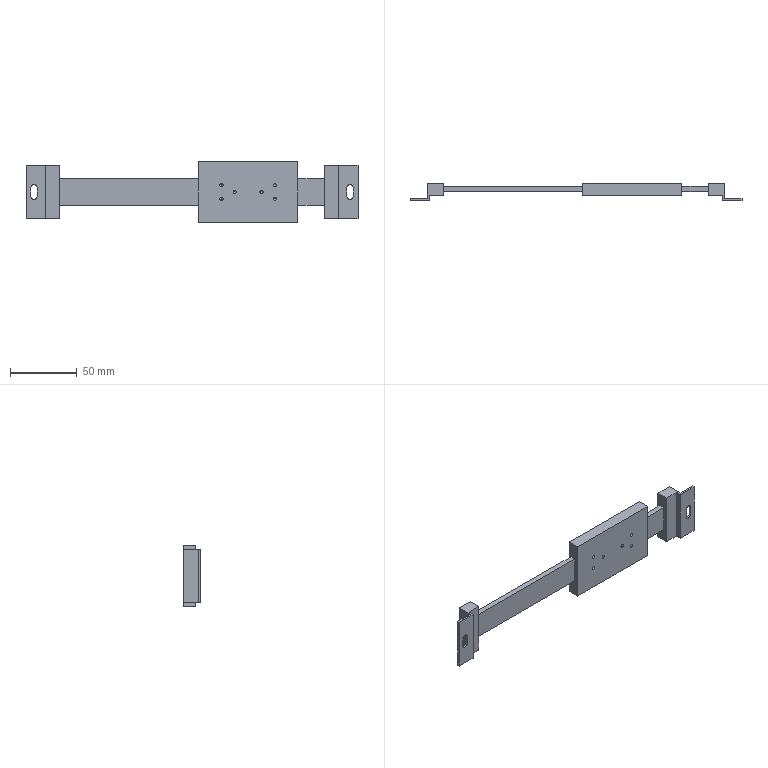Component | SolidWorks | CS021-DigitalScale-Range100-1 | 1 solid | 66 faces | box 248 x 13.25 x 45 mm | volume 50252 mm3 | plane 38 | cylinder 16 | cone 12 | commonest cylinder face diameters 2.5 x12 5 x4 | material AL6061
build123d program:
from build123d import *

# Parameters (mm, degrees)
SKETCH1_W                = 222
SKETCH1_H                = 20
BOSS_EXTRUDE1_DEPTH      = 2
BOSS_EXTRUDE2_DEPTH      = 20
CUT_EXTRUDE1_DEPTH       = 126.961
SKETCH4_W                = 40
SKETCH4_H                = 9
BOSS_EXTRUDE3_DEPTH      = 12
BOSS_EXTRUDE4_DEPTH      = 2
BOSS_EXTRUDE4_DEPTH_BACK = 7
SKETCH5_W                = 74
SKETCH5_H                = 45
M3_TAPPED_HOLE1_D        = 2.5
M3_TAPPED_HOLE1_DEPTH    = 6.5
M3_TAPPED_HOLE1_TIP      = 0.7511


with BuildPart() as part:
    # Sketch1 → Boss-Extrude1 (new, symmetric)
    with BuildSketch(Plane(origin=(0, 0, 0), x_dir=(1, 0, 0), z_dir=(0, 1, 0))):
        Rectangle(SKETCH1_W, SKETCH1_H)
    extrude(amount=BOSS_EXTRUDE1_DEPTH, both=True)

    # Sketch2 → Boss-Extrude2 (add, symmetric)
    with BuildSketch(Plane.XY):
        Polygon((-109.5, -2), (-109.5, -9), (-124, -9), (-124, -7.5), (-111, -7.5), (-111, -2), align=None)
    boss_extrude2 = extrude(amount=BOSS_EXTRUDE2_DEPTH, both=True)

    # Sketch3 → Cut-Extrude1 (cut, through all)
    with BuildSketch(Plane(origin=(0, -7.5, 0), x_dir=(1, 0, 0), z_dir=(0, 1, 0))):
        with BuildLine():
            Line((-115.5, 3), (-115.5, -3))
            ThreePointArc((-115.5, -3), (-118, -5.5), (-120.5, -3))
            Line((-120.5, -3), (-120.5, 3))
            ThreePointArc((-120.5, 3), (-118, 5.5), (-115.5, 3))
        make_face()
    cut_extrude1 = extrude(amount=-CUT_EXTRUDE1_DEPTH, mode=Mode.SUBTRACT)

    # Sketch4 → Boss-Extrude3 (add)
    with BuildSketch(Plane.ZY.offset(111)):
        with Locations((0, -0.25)):
            Rectangle(SKETCH4_W, SKETCH4_H)
    boss_extrude3 = extrude(amount=-BOSS_EXTRUDE3_DEPTH)

    # Mirror1: Boss-Extrude2, Cut-Extrude1, Boss-Extrude3 across plane
    add(boss_extrude2.mirror(Plane(origin=(0, 0, 0), x_dir=(0, 0, 1), z_dir=(1, 0, 0))))
    add(cut_extrude1.mirror(Plane(origin=(0, 0, 0), x_dir=(0, 0, 1), z_dir=(1, 0, 0))), mode=Mode.SUBTRACT)
    add(boss_extrude3.mirror(Plane(origin=(0, 0, 0), x_dir=(0, 0, 1), z_dir=(1, 0, 0))))

    # Sketch5 → Boss-Extrude4 (add, two sides: drawn at the far end of the back side and taken through both)
    with BuildSketch(Plane(origin=(0, 2, 0), x_dir=(1, 0, 0), z_dir=(0, 1, 0)).offset(-BOSS_EXTRUDE4_DEPTH_BACK)):
        with Locations((-42, 0)):
            Rectangle(SKETCH5_W, SKETCH5_H)
    extrude(amount=BOSS_EXTRUDE4_DEPTH + BOSS_EXTRUDE4_DEPTH_BACK)

    # M3 Tapped Hole1
    with Locations(Plane(origin=(0, -5, 0), x_dir=(-1, 0, 0), z_dir=(0, -1, 0))):
        with Locations((52, 0), (32, 0), (22, 5), (22, -5), (62, -5), (62, 5)):
            Hole(M3_TAPPED_HOLE1_D / 2, depth=M3_TAPPED_HOLE1_DEPTH)
            with Locations((0, 0, -(M3_TAPPED_HOLE1_DEPTH + M3_TAPPED_HOLE1_TIP / 2))):  # 118° drill point
                Cone(0, M3_TAPPED_HOLE1_D / 2, M3_TAPPED_HOLE1_TIP, mode=Mode.SUBTRACT)


solid = part.part

# Placed as in the assembly
solid = solid.moved(Location((110.449, 103.817, -85), (-180, 0, 180)))